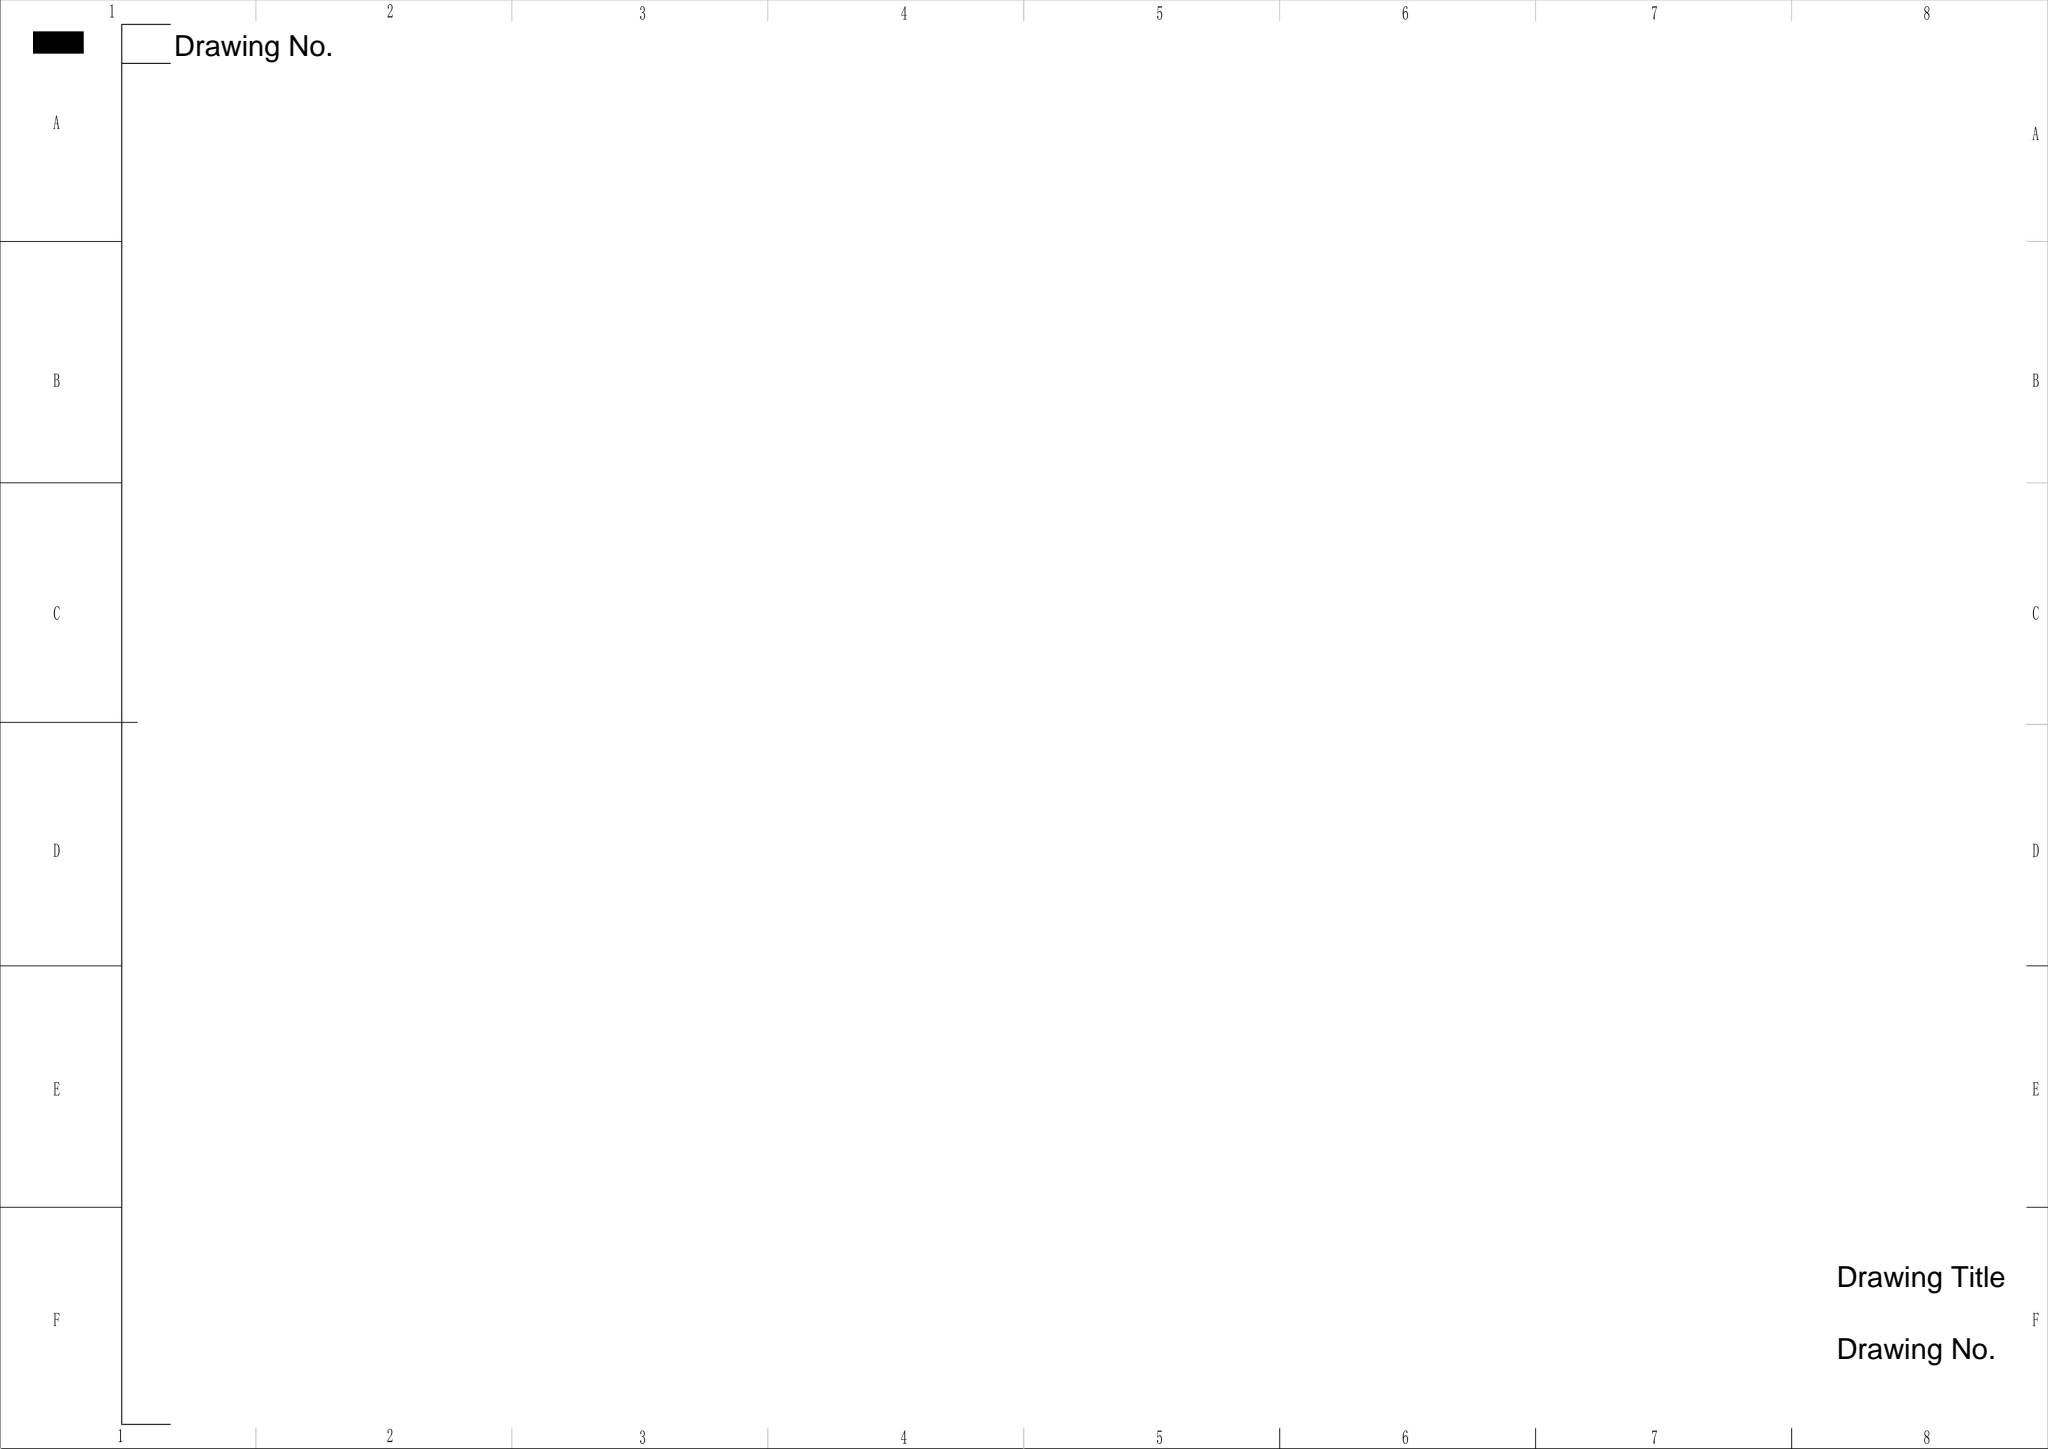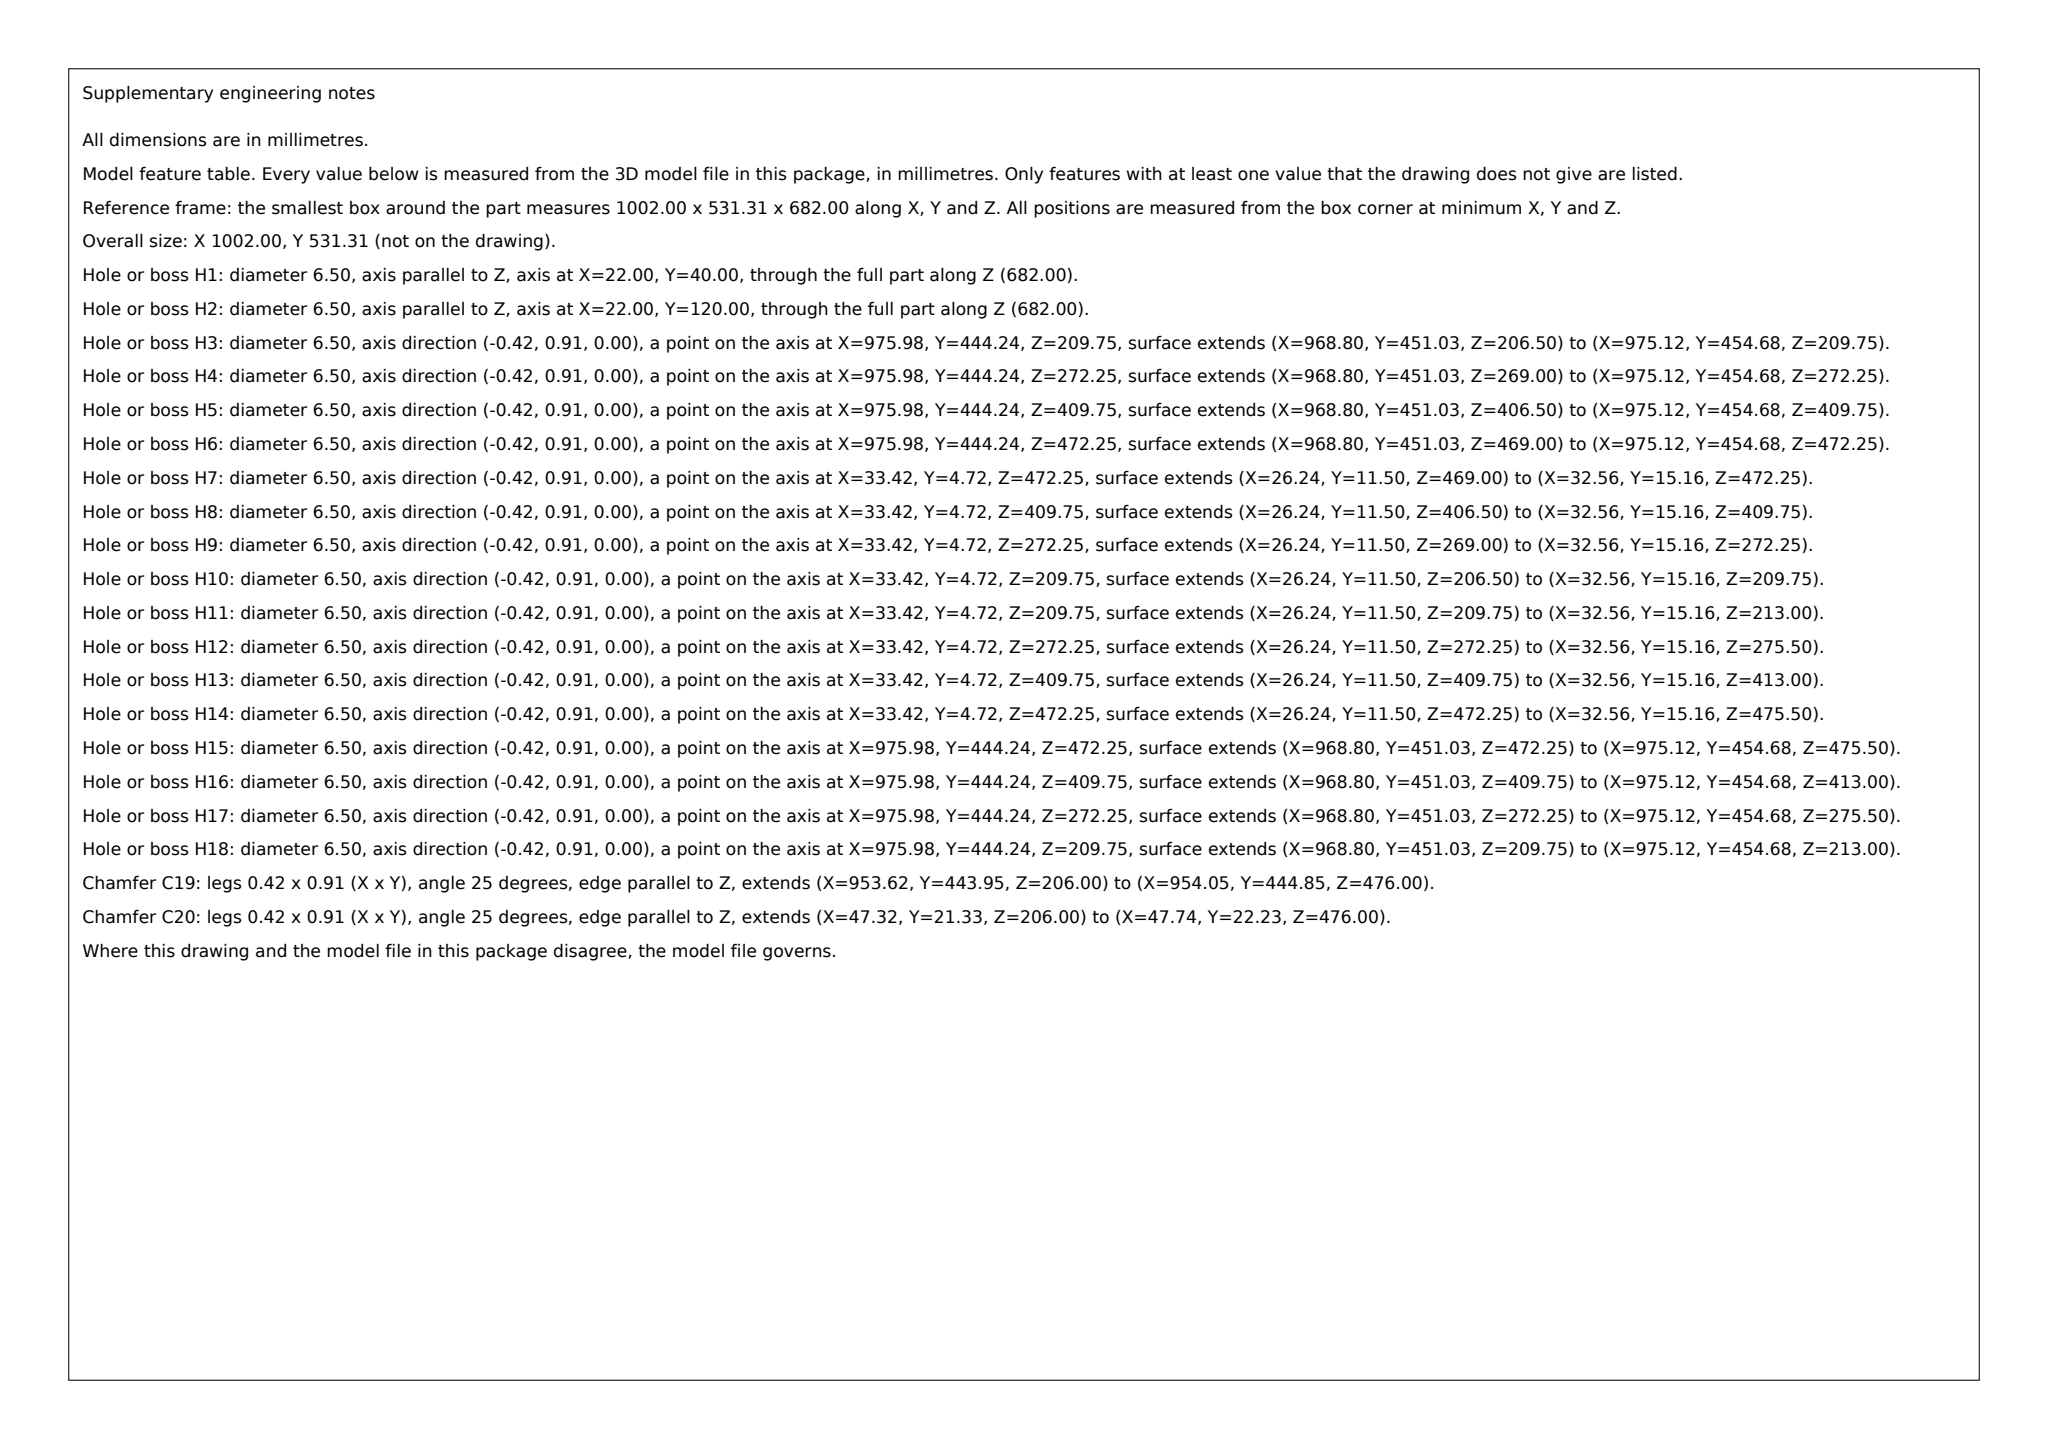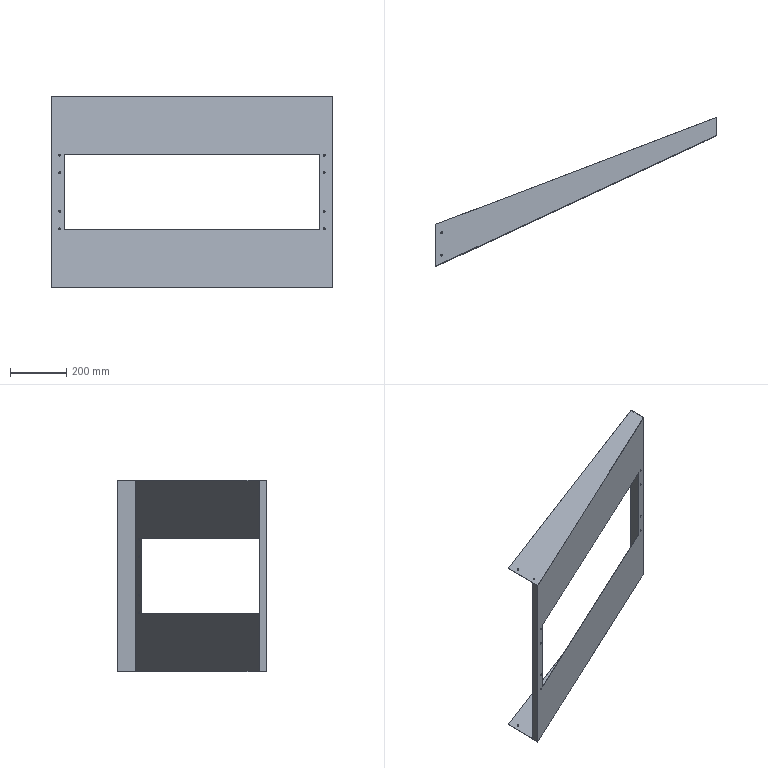Part | SolidWorks | mm | 1 solid | 43 faces | box 1002 x 531.31 x 682 mm | volume 773841 mm3 | cylinder 24 | plane 19 | commonest cylinder face diameters 6.5 x24